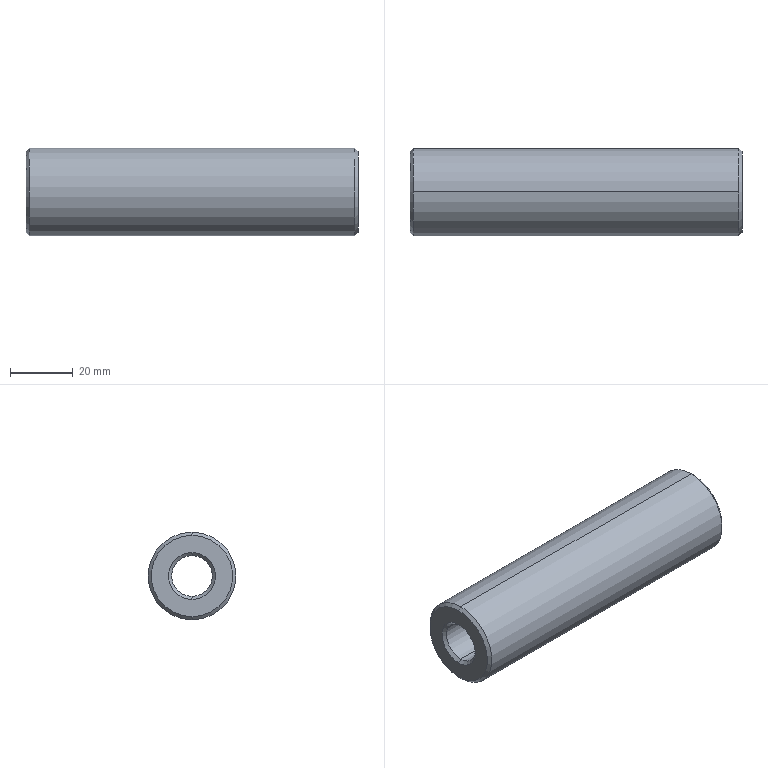Component | SolidWorks | LocatingGuideBushing106-2 | 1 solid | 14 faces | box 106 x 28 x 28 mm | volume 51071 mm3 | cone 8 | cylinder 4 | plane 2 | commonest cylinder face diameters 13 x2 28 x2
build123d program:
from build123d import *

# Parameters (mm, degrees)
SKETCH1_R           = 14
SKETCH1_R_2         = 6.5
BOSS_EXTRUDE1_DEPTH = 106
CHAMFER1_SIZE       = 1


with BuildPart() as part:
    # Sketch1 → Boss-Extrude1 (new body)
    with BuildSketch(Plane.XY):
        Circle(SKETCH1_R)
        Circle(SKETCH1_R_2, mode=Mode.SUBTRACT)
    extrude(amount=BOSS_EXTRUDE1_DEPTH)

    # Chamfer1
    chamfer1_edges = [part.edges().sort_by_distance(p)[0] for p in [
        (-14, 0, 0),
        (-14, 0, 106),
        (-6.5, 0, 0),
        (-6.5, 0, 106),
    ]]
    chamfer(chamfer1_edges, length=CHAMFER1_SIZE)


solid = part.part

# Placed as in the assembly
solid = solid.moved(Location((-45.809, -229.181, 0), (0, 90, 0)))
STEP:
#1=CARTESIAN_POINT('',(-1.804,-9.023,0.5118));
#2=VERTEX_POINT('',#1);
#3=CARTESIAN_POINT('',(-1.804,-9.023,-0.5118));
#4=VERTEX_POINT('',#3);
#5=CARTESIAN_POINT('',(-1.804,-9.023,-0.));
#6=DIRECTION('',(-1.,0.,-0.));
#7=DIRECTION('',(0.,0.,1.));
#8=AXIS2_PLACEMENT_3D('',#5,#6,#7);
#9=CIRCLE('',#8,0.5118);
#10=EDGE_CURVE('',#2,#4,#9,.T.);
#11=ORIENTED_EDGE('',*,*,#10,.F.);
#12=CARTESIAN_POINT('',(-1.764,-9.023,0.5512));
#13=VERTEX_POINT('',#12);
#14=CARTESIAN_POINT('',(-1.804,-9.023,0.5118));
#15=DIRECTION('',(0.7071,0.,0.7071));
#16=VECTOR('',#15,39.37);
#17=LINE('',#14,#16);
#18=EDGE_CURVE('',#2,#13,#17,.T.);
#19=ORIENTED_EDGE('',*,*,#18,.T.);
#20=CARTESIAN_POINT('',(-1.764,-9.023,-0.5512));
#21=VERTEX_POINT('',#20);
#22=CARTESIAN_POINT('',(-1.764,-9.023,-0.));
#23=DIRECTION('',(1.,-0.,0.));
#24=DIRECTION('',(0.,0.,1.));
#25=AXIS2_PLACEMENT_3D('',#22,#23,#24);
#26=CIRCLE('',#25,0.5512);
#27=EDGE_CURVE('',#21,#13,#26,.T.);
#28=ORIENTED_EDGE('',*,*,#27,.F.);
#29=CARTESIAN_POINT('',(-1.804,-9.023,-0.5118));
#30=DIRECTION('',(0.7071,-0.,-0.7071));
#31=VECTOR('',#30,39.37);
#32=LINE('',#29,#31);
#33=EDGE_CURVE('',#4,#21,#32,.T.);
#34=ORIENTED_EDGE('',*,*,#33,.F.);
#35=EDGE_LOOP('',(#11,#19,#28,#34));
#36=FACE_OUTER_BOUND('',#35,.T.);
#37=CARTESIAN_POINT('',(-1.804,-9.023,-0.));
#38=DIRECTION('',(1.,-0.,0.));
#39=DIRECTION('',(0.,0.,-1.));
#40=AXIS2_PLACEMENT_3D('',#37,#38,#39);
#41=CONICAL_SURFACE('',#40,0.5118,0.7854);
#42=ADVANCED_FACE('',(#36),#41,.T.);
#43=CARTESIAN_POINT('',(-1.764,-9.023,-0.2559));
#44=VERTEX_POINT('',#43);
#45=CARTESIAN_POINT('',(-1.764,-9.023,0.2559));
#46=VERTEX_POINT('',#45);
#47=CARTESIAN_POINT('',(-1.764,-9.023,-0.));
#48=DIRECTION('',(-1.,0.,-0.));
#49=DIRECTION('',(0.,0.,1.));
#50=AXIS2_PLACEMENT_3D('',#47,#48,#49);
#51=CIRCLE('',#50,0.2559);
#52=EDGE_CURVE('',#44,#46,#51,.T.);
#53=ORIENTED_EDGE('',*,*,#52,.F.);
#54=CARTESIAN_POINT('',(-1.804,-9.023,-0.2953));
#55=VERTEX_POINT('',#54);
#56=CARTESIAN_POINT('',(-1.764,-9.023,-0.2559));
#57=DIRECTION('',(-0.7071,0.,-0.7071));
#58=VECTOR('',#57,39.37);
#59=LINE('',#56,#58);
#60=EDGE_CURVE('',#44,#55,#59,.T.);
#61=ORIENTED_EDGE('',*,*,#60,.T.);
#62=CARTESIAN_POINT('',(-1.804,-9.023,0.2953));
#63=VERTEX_POINT('',#62);
#64=CARTESIAN_POINT('',(-1.804,-9.023,-0.));
#65=DIRECTION('',(1.,-0.,0.));
#66=DIRECTION('',(0.,0.,1.));
#67=AXIS2_PLACEMENT_3D('',#64,#65,#66);
#68=CIRCLE('',#67,0.2953);
#69=EDGE_CURVE('',#63,#55,#68,.T.);
#70=ORIENTED_EDGE('',*,*,#69,.F.);
#71=CARTESIAN_POINT('',(-1.764,-9.023,0.2559));
#72=DIRECTION('',(-0.7071,0.,0.7071));
#73=VECTOR('',#72,39.37);
#74=LINE('',#71,#73);
#75=EDGE_CURVE('',#46,#63,#74,.T.);
#76=ORIENTED_EDGE('',*,*,#75,.F.);
#77=EDGE_LOOP('',(#53,#61,#70,#76));
#78=FACE_OUTER_BOUND('',#77,.T.);
#79=CARTESIAN_POINT('',(-1.764,-9.023,-0.));
#80=DIRECTION('',(-1.,0.,-0.));
#81=DIRECTION('',(0.,0.,1.));
#82=AXIS2_PLACEMENT_3D('',#79,#80,#81);
#83=CONICAL_SURFACE('',#82,0.2559,0.7854);
#84=ADVANCED_FACE('',(#78),#83,.F.);
#85=CARTESIAN_POINT('',(2.37,-9.023,-0.5118));
#86=VERTEX_POINT('',#85);
#87=CARTESIAN_POINT('',(2.37,-9.023,0.5118));
#88=VERTEX_POINT('',#87);
#89=CARTESIAN_POINT('',(2.37,-9.023,-0.));
#90=DIRECTION('',(1.,-0.,0.));
#91=DIRECTION('',(0.,0.,1.));
#92=AXIS2_PLACEMENT_3D('',#89,#90,#91);
#93=CIRCLE('',#92,0.5118);
#94=EDGE_CURVE('',#86,#88,#93,.T.);
#95=ORIENTED_EDGE('',*,*,#94,.F.);
#96=CARTESIAN_POINT('',(2.33,-9.023,-0.5512));
#97=VERTEX_POINT('',#96);
#98=CARTESIAN_POINT('',(2.33,-9.023,-0.5512));
#99=DIRECTION('',(-0.7071,0.,-0.7071));
#100=VECTOR('',#99,39.37);
#101=LINE('',#98,#100);
#102=EDGE_CURVE('',#86,#97,#101,.T.);
#103=ORIENTED_EDGE('',*,*,#102,.T.);
#104=CARTESIAN_POINT('',(2.33,-9.023,0.5512));
#105=VERTEX_POINT('',#104);
#106=CARTESIAN_POINT('',(2.33,-9.023,-0.));
#107=DIRECTION('',(-1.,0.,-0.));
#108=DIRECTION('',(0.,0.,1.));
#109=AXIS2_PLACEMENT_3D('',#106,#107,#108);
#110=CIRCLE('',#109,0.5512);
#111=EDGE_CURVE('',#105,#97,#110,.T.);
#112=ORIENTED_EDGE('',*,*,#111,.F.);
#113=CARTESIAN_POINT('',(2.33,-9.023,0.5512));
#114=DIRECTION('',(-0.7071,0.,0.7071));
#115=VECTOR('',#114,39.37);
#116=LINE('',#113,#115);
#117=EDGE_CURVE('',#88,#105,#116,.T.);
#118=ORIENTED_EDGE('',*,*,#117,.F.);
#119=EDGE_LOOP('',(#95,#103,#112,#118));
#120=FACE_OUTER_BOUND('',#119,.T.);
#121=CARTESIAN_POINT('',(2.33,-9.023,-0.));
#122=DIRECTION('',(-1.,0.,-0.));
#123=DIRECTION('',(0.,0.,1.));
#124=AXIS2_PLACEMENT_3D('',#121,#122,#123);
#125=CONICAL_SURFACE('',#124,0.5512,0.7854);
#126=ADVANCED_FACE('',(#120),#125,.T.);
#127=CARTESIAN_POINT('',(2.33,-9.023,0.2559));
#128=VERTEX_POINT('',#127);
#129=CARTESIAN_POINT('',(2.33,-9.023,-0.2559));
#130=VERTEX_POINT('',#129);
#131=CARTESIAN_POINT('',(2.33,-9.023,-0.));
#132=DIRECTION('',(1.,-0.,0.));
#133=DIRECTION('',(0.,0.,1.));
#134=AXIS2_PLACEMENT_3D('',#131,#132,#133);
#135=CIRCLE('',#134,0.2559);
#136=EDGE_CURVE('',#128,#130,#135,.T.);
#137=ORIENTED_EDGE('',*,*,#136,.F.);
#138=CARTESIAN_POINT('',(2.37,-9.023,0.2953));
#139=VERTEX_POINT('',#138);
#140=CARTESIAN_POINT('',(2.37,-9.023,0.2953));
#141=DIRECTION('',(0.7071,0.,0.7071));
#142=VECTOR('',#141,39.37);
#143=LINE('',#140,#142);
#144=EDGE_CURVE('',#128,#139,#143,.T.);
#145=ORIENTED_EDGE('',*,*,#144,.T.);
#146=CARTESIAN_POINT('',(2.37,-9.023,-0.2953));
#147=VERTEX_POINT('',#146);
#148=CARTESIAN_POINT('',(2.37,-9.023,-0.));
#149=DIRECTION('',(-1.,0.,-0.));
#150=DIRECTION('',(0.,0.,1.));
#151=AXIS2_PLACEMENT_3D('',#148,#149,#150);
#152=CIRCLE('',#151,0.2953);
#153=EDGE_CURVE('',#147,#139,#152,.T.);
#154=ORIENTED_EDGE('',*,*,#153,.F.);
#155=CARTESIAN_POINT('',(2.37,-9.023,-0.2953));
#156=DIRECTION('',(0.7071,-0.,-0.7071));
#157=VECTOR('',#156,39.37);
#158=LINE('',#155,#157);
#159=EDGE_CURVE('',#130,#147,#158,.T.);
#160=ORIENTED_EDGE('',*,*,#159,.F.);
#161=EDGE_LOOP('',(#137,#145,#154,#160));
#162=FACE_OUTER_BOUND('',#161,.T.);
#163=CARTESIAN_POINT('',(2.37,-9.023,-0.));
#164=DIRECTION('',(1.,-0.,0.));
#165=DIRECTION('',(0.,0.,-1.));
#166=AXIS2_PLACEMENT_3D('',#163,#164,#165);
#167=CONICAL_SURFACE('',#166,0.2953,0.7854);
#168=ADVANCED_FACE('',(#162),#167,.F.);
#169=ORIENTED_EDGE('',*,*,#52,.T.);
#170=CARTESIAN_POINT('',(-1.804,-9.023,0.2559));
#171=DIRECTION('',(1.,-0.,0.));
#172=VECTOR('',#171,39.37);
#173=LINE('',#170,#172);
#174=EDGE_CURVE('',#46,#128,#173,.T.);
#175=ORIENTED_EDGE('',*,*,#174,.T.);
#176=ORIENTED_EDGE('',*,*,#136,.T.);
#177=CARTESIAN_POINT('',(-1.804,-9.023,-0.2559));
#178=DIRECTION('',(1.,-0.,0.));
#179=VECTOR('',#178,39.37);
#180=LINE('',#177,#179);
#181=EDGE_CURVE('',#44,#130,#180,.T.);
#182=ORIENTED_EDGE('',*,*,#181,.F.);
#183=EDGE_LOOP('',(#169,#175,#176,#182));
#184=FACE_OUTER_BOUND('',#183,.T.);
#185=CARTESIAN_POINT('',(-1.804,-9.023,-0.));
#186=DIRECTION('',(1.,-0.,0.));
#187=DIRECTION('',(0.,0.,-1.));
#188=AXIS2_PLACEMENT_3D('',#185,#186,#187);
#189=CYLINDRICAL_SURFACE('',#188,0.2559);
#190=ADVANCED_FACE('',(#184),#189,.F.);
#191=ORIENTED_EDGE('',*,*,#27,.T.);
#192=CARTESIAN_POINT('',(-1.804,-9.023,0.5512));
#193=DIRECTION('',(1.,-0.,0.));
#194=VECTOR('',#193,39.37);
#195=LINE('',#192,#194);
#196=EDGE_CURVE('',#13,#105,#195,.T.);
#197=ORIENTED_EDGE('',*,*,#196,.T.);
#198=ORIENTED_EDGE('',*,*,#111,.T.);
#199=CARTESIAN_POINT('',(-1.804,-9.023,-0.5512));
#200=DIRECTION('',(1.,-0.,0.));
#201=VECTOR('',#200,39.37);
#202=LINE('',#199,#201);
#203=EDGE_CURVE('',#21,#97,#202,.T.);
#204=ORIENTED_EDGE('',*,*,#203,.F.);
#205=EDGE_LOOP('',(#191,#197,#198,#204));
#206=FACE_OUTER_BOUND('',#205,.T.);
#207=CARTESIAN_POINT('',(-1.804,-9.023,-0.));
#208=DIRECTION('',(1.,-0.,0.));
#209=DIRECTION('',(0.,0.,-1.));
#210=AXIS2_PLACEMENT_3D('',#207,#208,#209);
#211=CYLINDRICAL_SURFACE('',#210,0.5512);
#212=ADVANCED_FACE('',(#206),#211,.T.);
#213=ORIENTED_EDGE('',*,*,#69,.T.);
#214=CARTESIAN_POINT('',(-1.804,-9.023,-0.));
#215=DIRECTION('',(1.,-0.,0.));
#216=DIRECTION('',(0.,0.,1.));
#217=AXIS2_PLACEMENT_3D('',#214,#215,#216);
#218=CIRCLE('',#217,0.2953);
#219=EDGE_CURVE('',#55,#63,#218,.T.);
#220=ORIENTED_EDGE('',*,*,#219,.T.);
#221=EDGE_LOOP('',(#213,#220));
#222=FACE_BOUND('',#221,.T.);
#223=CARTESIAN_POINT('',(-1.804,-9.023,-0.));
#224=DIRECTION('',(-1.,0.,-0.));
#225=DIRECTION('',(0.,0.,1.));
#226=AXIS2_PLACEMENT_3D('',#223,#224,#225);
#227=CIRCLE('',#226,0.5118);
#228=EDGE_CURVE('',#4,#2,#227,.T.);
#229=ORIENTED_EDGE('',*,*,#228,.T.);
#230=ORIENTED_EDGE('',*,*,#10,.T.);
#231=EDGE_LOOP('',(#229,#230));
#232=FACE_OUTER_BOUND('',#231,.T.);
#233=CARTESIAN_POINT('',(-1.804,-9.023,-0.));
#234=DIRECTION('',(-1.,0.,-0.));
#235=DIRECTION('',(-0.,0.,1.));
#236=AXIS2_PLACEMENT_3D('',#233,#234,#235);
#237=PLANE('',#236);
#238=ADVANCED_FACE('',(#222,#232),#237,.T.);
#239=ORIENTED_EDGE('',*,*,#153,.T.);
#240=CARTESIAN_POINT('',(2.37,-9.023,-0.));
#241=DIRECTION('',(-1.,0.,-0.));
#242=DIRECTION('',(0.,0.,1.));
#243=AXIS2_PLACEMENT_3D('',#240,#241,#242);
#244=CIRCLE('',#243,0.2953);
#245=EDGE_CURVE('',#139,#147,#244,.T.);
#246=ORIENTED_EDGE('',*,*,#245,.T.);
#247=EDGE_LOOP('',(#239,#246));
#248=FACE_BOUND('',#247,.T.);
#249=CARTESIAN_POINT('',(2.37,-9.023,-0.));
#250=DIRECTION('',(1.,-0.,0.));
#251=DIRECTION('',(0.,0.,1.));
#252=AXIS2_PLACEMENT_3D('',#249,#250,#251);
#253=CIRCLE('',#252,0.5118);
#254=EDGE_CURVE('',#88,#86,#253,.T.);
#255=ORIENTED_EDGE('',*,*,#254,.T.);
#256=ORIENTED_EDGE('',*,*,#94,.T.);
#257=EDGE_LOOP('',(#255,#256));
#258=FACE_OUTER_BOUND('',#257,.T.);
#259=CARTESIAN_POINT('',(2.37,-9.023,-0.));
#260=DIRECTION('',(-1.,0.,-0.));
#261=DIRECTION('',(-0.,0.,1.));
#262=AXIS2_PLACEMENT_3D('',#259,#260,#261);
#263=PLANE('',#262);
#264=ADVANCED_FACE('',(#248,#258),#263,.F.);
#265=ORIENTED_EDGE('',*,*,#196,.F.);
#266=CARTESIAN_POINT('',(-1.764,-9.023,-0.));
#267=DIRECTION('',(1.,-0.,0.));
#268=DIRECTION('',(0.,-0.,1.));
#269=AXIS2_PLACEMENT_3D('',#266,#267,#268);
#270=CIRCLE('',#269,0.5512);
#271=EDGE_CURVE('',#13,#21,#270,.T.);
#272=ORIENTED_EDGE('',*,*,#271,.T.);
#273=ORIENTED_EDGE('',*,*,#203,.T.);
#274=CARTESIAN_POINT('',(2.33,-9.023,-0.));
#275=DIRECTION('',(-1.,0.,-0.));
#276=DIRECTION('',(0.,0.,1.));
#277=AXIS2_PLACEMENT_3D('',#274,#275,#276);
#278=CIRCLE('',#277,0.5512);
#279=EDGE_CURVE('',#97,#105,#278,.T.);
#280=ORIENTED_EDGE('',*,*,#279,.T.);
#281=EDGE_LOOP('',(#265,#272,#273,#280));
#282=FACE_OUTER_BOUND('',#281,.T.);
#283=CARTESIAN_POINT('',(-1.804,-9.023,-0.));
#284=DIRECTION('',(1.,-0.,0.));
#285=DIRECTION('',(0.,0.,-1.));
#286=AXIS2_PLACEMENT_3D('',#283,#284,#285);
#287=CYLINDRICAL_SURFACE('',#286,0.5512);
#288=ADVANCED_FACE('',(#282),#287,.T.);
#289=ORIENTED_EDGE('',*,*,#174,.F.);
#290=CARTESIAN_POINT('',(-1.764,-9.023,-0.));
#291=DIRECTION('',(-1.,0.,-0.));
#292=DIRECTION('',(0.,0.,1.));
#293=AXIS2_PLACEMENT_3D('',#290,#291,#292);
#294=CIRCLE('',#293,0.2559);
#295=EDGE_CURVE('',#46,#44,#294,.T.);
#296=ORIENTED_EDGE('',*,*,#295,.T.);
#297=ORIENTED_EDGE('',*,*,#181,.T.);
#298=CARTESIAN_POINT('',(2.33,-9.023,-0.));
#299=DIRECTION('',(1.,-0.,0.));
#300=DIRECTION('',(0.,0.,1.));
#301=AXIS2_PLACEMENT_3D('',#298,#299,#300);
#302=CIRCLE('',#301,0.2559);
#303=EDGE_CURVE('',#130,#128,#302,.T.);
#304=ORIENTED_EDGE('',*,*,#303,.T.);
#305=EDGE_LOOP('',(#289,#296,#297,#304));
#306=FACE_OUTER_BOUND('',#305,.T.);
#307=CARTESIAN_POINT('',(-1.804,-9.023,-0.));
#308=DIRECTION('',(1.,-0.,0.));
#309=DIRECTION('',(0.,0.,-1.));
#310=AXIS2_PLACEMENT_3D('',#307,#308,#309);
#311=CYLINDRICAL_SURFACE('',#310,0.2559);
#312=ADVANCED_FACE('',(#306),#311,.F.);
#313=ORIENTED_EDGE('',*,*,#144,.F.);
#314=ORIENTED_EDGE('',*,*,#303,.F.);
#315=ORIENTED_EDGE('',*,*,#159,.T.);
#316=ORIENTED_EDGE('',*,*,#245,.F.);
#317=EDGE_LOOP('',(#313,#314,#315,#316));
#318=FACE_OUTER_BOUND('',#317,.T.);
#319=CARTESIAN_POINT('',(2.37,-9.023,-0.));
#320=DIRECTION('',(1.,-0.,0.));
#321=DIRECTION('',(0.,0.,-1.));
#322=AXIS2_PLACEMENT_3D('',#319,#320,#321);
#323=CONICAL_SURFACE('',#322,0.2953,0.7854);
#324=ADVANCED_FACE('',(#318),#323,.F.);
#325=ORIENTED_EDGE('',*,*,#102,.F.);
#326=ORIENTED_EDGE('',*,*,#254,.F.);
#327=ORIENTED_EDGE('',*,*,#117,.T.);
#328=ORIENTED_EDGE('',*,*,#279,.F.);
#329=EDGE_LOOP('',(#325,#326,#327,#328));
#330=FACE_OUTER_BOUND('',#329,.T.);
#331=CARTESIAN_POINT('',(2.33,-9.023,-0.));
#332=DIRECTION('',(-1.,0.,-0.));
#333=DIRECTION('',(0.,0.,1.));
#334=AXIS2_PLACEMENT_3D('',#331,#332,#333);
#335=CONICAL_SURFACE('',#334,0.5512,0.7854);
#336=ADVANCED_FACE('',(#330),#335,.T.);
#337=ORIENTED_EDGE('',*,*,#60,.F.);
#338=ORIENTED_EDGE('',*,*,#295,.F.);
#339=ORIENTED_EDGE('',*,*,#75,.T.);
#340=ORIENTED_EDGE('',*,*,#219,.F.);
#341=EDGE_LOOP('',(#337,#338,#339,#340));
#342=FACE_OUTER_BOUND('',#341,.T.);
#343=CARTESIAN_POINT('',(-1.764,-9.023,-0.));
#344=DIRECTION('',(-1.,0.,-0.));
#345=DIRECTION('',(0.,0.,1.));
#346=AXIS2_PLACEMENT_3D('',#343,#344,#345);
#347=CONICAL_SURFACE('',#346,0.2559,0.7854);
#348=ADVANCED_FACE('',(#342),#347,.F.);
#349=ORIENTED_EDGE('',*,*,#18,.F.);
#350=ORIENTED_EDGE('',*,*,#228,.F.);
#351=ORIENTED_EDGE('',*,*,#33,.T.);
#352=ORIENTED_EDGE('',*,*,#271,.F.);
#353=EDGE_LOOP('',(#349,#350,#351,#352));
#354=FACE_OUTER_BOUND('',#353,.T.);
#355=CARTESIAN_POINT('',(-1.804,-9.023,-0.));
#356=DIRECTION('',(1.,-0.,0.));
#357=DIRECTION('',(0.,0.,-1.));
#358=AXIS2_PLACEMENT_3D('',#355,#356,#357);
#359=CONICAL_SURFACE('',#358,0.5118,0.7854);
#360=ADVANCED_FACE('',(#354),#359,.T.);
#361=CLOSED_SHELL('',(#42,#84,#126,#168,#190,#212,#238,#264,#288,#312,#324,#336,#348,#360));
#362=MANIFOLD_SOLID_BREP('',#361);
#363=CARTESIAN_POINT('',(0.,0.,0.));
#364=DIRECTION('',(0.,0.,1.));
#365=DIRECTION('',(1.,0.,0.));
#366=AXIS2_PLACEMENT_3D('',#363,#364,#365);
#367=(LENGTH_UNIT()NAMED_UNIT(*)SI_UNIT($,.METRE.));
#368=LENGTH_MEASURE_WITH_UNIT(LENGTH_MEASURE(0.0254),#367);
#369=DIMENSIONAL_EXPONENTS(1.,0.,0.,0.,0.,0.,0.);
#370=(CONVERSION_BASED_UNIT('',#368)LENGTH_UNIT()NAMED_UNIT(#369));
#371=UNCERTAINTY_MEASURE_WITH_UNIT(LENGTH_MEASURE(0.00001),#370,'','');
#372=(NAMED_UNIT(*)PLANE_ANGLE_UNIT()SI_UNIT($,.RADIAN.));
#373=(NAMED_UNIT(*)SI_UNIT($,.STERADIAN.)SOLID_ANGLE_UNIT());
#374=(GEOMETRIC_REPRESENTATION_CONTEXT(3)GLOBAL_UNCERTAINTY_ASSIGNED_CONTEXT((#371))GLOBAL_UNIT_ASSIGNED_CONTEXT((#370,#372,#373))REPRESENTATION_CONTEXT('',''));
#375=ADVANCED_BREP_SHAPE_REPRESENTATION('',(#362,#366),#374);
#376=COLOUR_RGB('',0.7922,0.8196,0.9333);
#377=FILL_AREA_STYLE_COLOUR('',#376);
#378=FILL_AREA_STYLE('',(#377));
#379=SURFACE_STYLE_FILL_AREA(#378);
#380=SURFACE_SIDE_STYLE('',(#379));
#381=SURFACE_STYLE_USAGE(.BOTH.,#380);
#382=PRESENTATION_STYLE_ASSIGNMENT((#381));
#383=STYLED_ITEM('',(#382),#362);
#384=(LENGTH_UNIT()NAMED_UNIT(*)SI_UNIT($,.METRE.));
#385=LENGTH_MEASURE_WITH_UNIT(LENGTH_MEASURE(0.0254),#384);
#386=DIMENSIONAL_EXPONENTS(1.,0.,0.,0.,0.,0.,0.);
#387=(CONVERSION_BASED_UNIT('',#385)LENGTH_UNIT()NAMED_UNIT(#386));
#388=UNCERTAINTY_MEASURE_WITH_UNIT(LENGTH_MEASURE(0.00001),#387,'','');
#389=(NAMED_UNIT(*)PLANE_ANGLE_UNIT()SI_UNIT($,.RADIAN.));
#390=(NAMED_UNIT(*)SI_UNIT($,.STERADIAN.)SOLID_ANGLE_UNIT());
#391=(GEOMETRIC_REPRESENTATION_CONTEXT(3)GLOBAL_UNCERTAINTY_ASSIGNED_CONTEXT((#388))GLOBAL_UNIT_ASSIGNED_CONTEXT((#387,#389,#390))REPRESENTATION_CONTEXT('',''));
#392=MECHANICAL_DESIGN_GEOMETRIC_PRESENTATION_REPRESENTATION('',(#383),#391);
#393=PRESENTATION_LAYER_ASSIGNMENT('','',(#383));